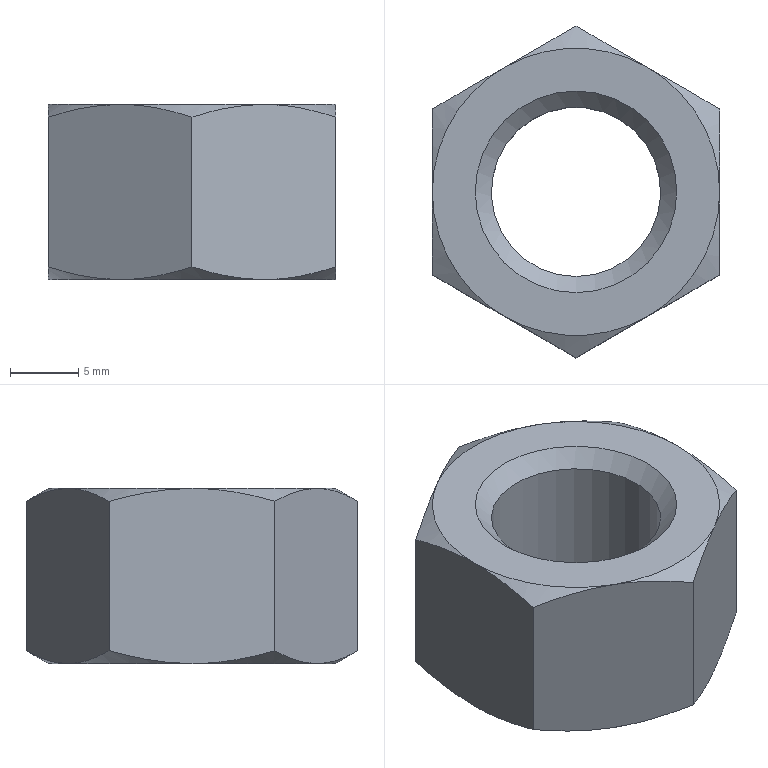Component | NX | GB-T6170_F-2000_M14X2 | 1 solid | 23 faces | volume 3271 mm3 | cone 14 | plane 8 | cylinder 1 | commonest cylinder face diameters 12.376 x1